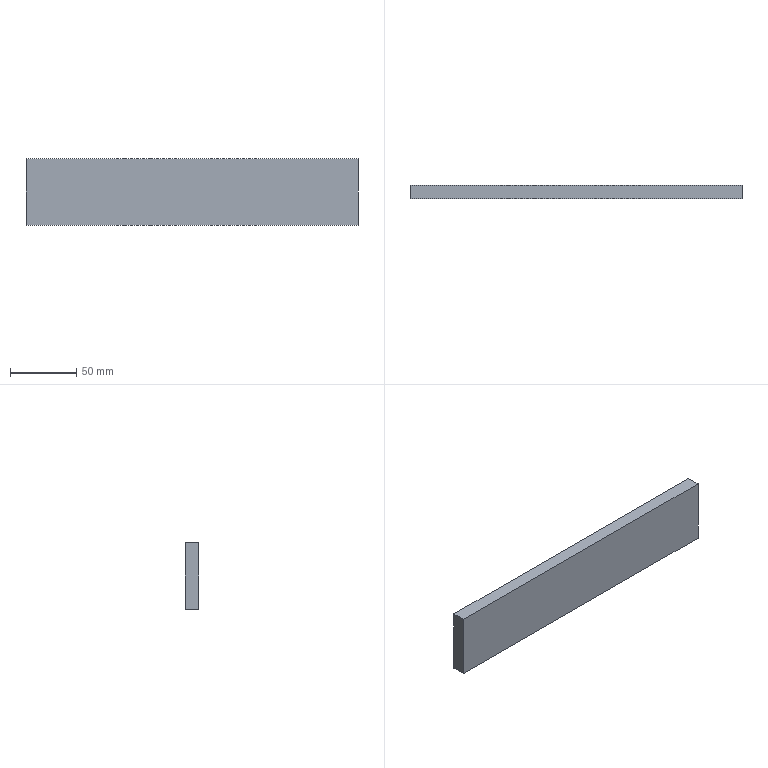Component | NX | FRONT_BLOCK | 1 solid | 6 faces | box 250 x 10 x 50 mm | volume 125000 mm3 | plane 6
STEP:
#1=CARTESIAN_POINT('',(0.,0.,0.));
#2=DIRECTION('',(0.,0.,1.));
#3=DIRECTION('',(1.,0.,0.));
#4=AXIS2_PLACEMENT_3D('',#1,#2,#3);
#5=CARTESIAN_POINT('',(280.662,80.,-20.));
#6=VERTEX_POINT('',#5);
#7=CARTESIAN_POINT('',(280.662,80.,30.));
#8=VERTEX_POINT('',#7);
#9=CARTESIAN_POINT('',(280.662,80.,-20.));
#10=DIRECTION('',(-0.,0.,1.));
#11=VECTOR('',#10,1.);
#12=LINE('',#9,#11);
#13=CARTESIAN_POINT('',(280.662,90.,-20.));
#14=DIRECTION('',(1.,0.,0.));
#15=DIRECTION('',(0.,0.,-1.));
#16=AXIS2_PLACEMENT_3D('',#13,#14,#15);
#17=PLANE('',#16);
#18=CARTESIAN_POINT('',(0.,-10.));
#19=DIRECTION('',(-1.,0.));
#20=VECTOR('',#19,1.);
#21=LINE('',#18,#20);
#22=(GEOMETRIC_REPRESENTATION_CONTEXT(2)PARAMETRIC_REPRESENTATION_CONTEXT()REPRESENTATION_CONTEXT('',''));
#23=DEFINITIONAL_REPRESENTATION('',(#21),#22);
#24=PCURVE('',#17,#23);
#25=CARTESIAN_POINT('',(280.662,80.,-20.));
#26=DIRECTION('',(0.,1.,0.));
#27=DIRECTION('',(1.,0.,0.));
#28=AXIS2_PLACEMENT_3D('',#25,#26,#27);
#29=PLANE('',#28);
#30=CARTESIAN_POINT('',(0.,0.));
#31=DIRECTION('',(-0.,-1.));
#32=VECTOR('',#31,1.);
#33=LINE('',#30,#32);
#34=(GEOMETRIC_REPRESENTATION_CONTEXT(2)PARAMETRIC_REPRESENTATION_CONTEXT()REPRESENTATION_CONTEXT('',''));
#35=DEFINITIONAL_REPRESENTATION('',(#33),#34);
#36=PCURVE('',#29,#35);
#37=SURFACE_CURVE('',#12,(#24,#36),.PCURVE_S1.);
#38=EDGE_CURVE('',#6,#8,#37,.T.);
#39=ORIENTED_EDGE('',*,*,#38,.T.);
#40=CARTESIAN_POINT('',(280.662,90.,30.));
#41=VERTEX_POINT('',#40);
#42=CARTESIAN_POINT('',(280.662,90.,30.));
#43=DIRECTION('',(0.,-1.,0.));
#44=VECTOR('',#43,1.);
#45=LINE('',#42,#44);
#46=CARTESIAN_POINT('',(-50.,0.));
#47=DIRECTION('',(0.,-1.));
#48=VECTOR('',#47,1.);
#49=LINE('',#46,#48);
#50=(GEOMETRIC_REPRESENTATION_CONTEXT(2)PARAMETRIC_REPRESENTATION_CONTEXT()REPRESENTATION_CONTEXT('',''));
#51=DEFINITIONAL_REPRESENTATION('',(#49),#50);
#52=PCURVE('',#17,#51);
#53=CARTESIAN_POINT('',(280.662,90.,30.));
#54=DIRECTION('',(0.,0.,-1.));
#55=DIRECTION('',(0.,1.,0.));
#56=AXIS2_PLACEMENT_3D('',#53,#54,#55);
#57=PLANE('',#56);
#58=CARTESIAN_POINT('',(0.,0.));
#59=DIRECTION('',(-1.,0.));
#60=VECTOR('',#59,1.);
#61=LINE('',#58,#60);
#62=(GEOMETRIC_REPRESENTATION_CONTEXT(2)PARAMETRIC_REPRESENTATION_CONTEXT()REPRESENTATION_CONTEXT('',''));
#63=DEFINITIONAL_REPRESENTATION('',(#61),#62);
#64=PCURVE('',#57,#63);
#65=SURFACE_CURVE('',#45,(#52,#64),.PCURVE_S1.);
#66=EDGE_CURVE('',#41,#8,#65,.T.);
#67=ORIENTED_EDGE('',*,*,#66,.F.);
#68=CARTESIAN_POINT('',(280.662,90.,-20.));
#69=VERTEX_POINT('',#68);
#70=CARTESIAN_POINT('',(280.662,90.,-20.));
#71=DIRECTION('',(-0.,0.,1.));
#72=VECTOR('',#71,1.);
#73=LINE('',#70,#72);
#74=CARTESIAN_POINT('',(0.,0.));
#75=DIRECTION('',(-1.,0.));
#76=VECTOR('',#75,1.);
#77=LINE('',#74,#76);
#78=(GEOMETRIC_REPRESENTATION_CONTEXT(2)PARAMETRIC_REPRESENTATION_CONTEXT()REPRESENTATION_CONTEXT('',''));
#79=DEFINITIONAL_REPRESENTATION('',(#77),#78);
#80=PCURVE('',#17,#79);
#81=CARTESIAN_POINT('',(280.662,90.,-20.));
#82=DIRECTION('',(0.,1.,0.));
#83=DIRECTION('',(1.,0.,0.));
#84=AXIS2_PLACEMENT_3D('',#81,#82,#83);
#85=PLANE('',#84);
#86=CARTESIAN_POINT('',(0.,0.));
#87=DIRECTION('',(-0.,-1.));
#88=VECTOR('',#87,1.);
#89=LINE('',#86,#88);
#90=(GEOMETRIC_REPRESENTATION_CONTEXT(2)PARAMETRIC_REPRESENTATION_CONTEXT()REPRESENTATION_CONTEXT('',''));
#91=DEFINITIONAL_REPRESENTATION('',(#89),#90);
#92=PCURVE('',#85,#91);
#93=SURFACE_CURVE('',#73,(#80,#92),.PCURVE_S1.);
#94=EDGE_CURVE('',#69,#41,#93,.T.);
#95=ORIENTED_EDGE('',*,*,#94,.F.);
#96=CARTESIAN_POINT('',(280.662,90.,-20.));
#97=DIRECTION('',(0.,-1.,0.));
#98=VECTOR('',#97,1.);
#99=LINE('',#96,#98);
#100=CARTESIAN_POINT('',(0.,0.));
#101=DIRECTION('',(0.,-1.));
#102=VECTOR('',#101,1.);
#103=LINE('',#100,#102);
#104=(GEOMETRIC_REPRESENTATION_CONTEXT(2)PARAMETRIC_REPRESENTATION_CONTEXT()REPRESENTATION_CONTEXT('',''));
#105=DEFINITIONAL_REPRESENTATION('',(#103),#104);
#106=PCURVE('',#17,#105);
#107=CARTESIAN_POINT('',(530.662,90.,-20.));
#108=DIRECTION('',(0.,0.,1.));
#109=DIRECTION('',(0.,-1.,0.));
#110=AXIS2_PLACEMENT_3D('',#107,#108,#109);
#111=PLANE('',#110);
#112=CARTESIAN_POINT('',(0.,-250.));
#113=DIRECTION('',(1.,0.));
#114=VECTOR('',#113,1.);
#115=LINE('',#112,#114);
#116=(GEOMETRIC_REPRESENTATION_CONTEXT(2)PARAMETRIC_REPRESENTATION_CONTEXT()REPRESENTATION_CONTEXT('',''));
#117=DEFINITIONAL_REPRESENTATION('',(#115),#116);
#118=PCURVE('',#111,#117);
#119=SURFACE_CURVE('',#99,(#106,#118),.PCURVE_S1.);
#120=EDGE_CURVE('',#69,#6,#119,.T.);
#121=ORIENTED_EDGE('',*,*,#120,.T.);
#122=EDGE_LOOP('',(#39,#67,#95,#121));
#123=FACE_BOUND('',#122,.T.);
#124=ADVANCED_FACE('',(#123),#17,.F.);
#125=CARTESIAN_POINT('',(530.662,80.,30.));
#126=VERTEX_POINT('',#125);
#127=CARTESIAN_POINT('',(280.662,80.,30.));
#128=DIRECTION('',(1.,0.,0.));
#129=VECTOR('',#128,1.);
#130=LINE('',#127,#129);
#131=CARTESIAN_POINT('',(-10.,0.));
#132=DIRECTION('',(0.,1.));
#133=VECTOR('',#132,1.);
#134=LINE('',#131,#133);
#135=(GEOMETRIC_REPRESENTATION_CONTEXT(2)PARAMETRIC_REPRESENTATION_CONTEXT()REPRESENTATION_CONTEXT('',''));
#136=DEFINITIONAL_REPRESENTATION('',(#134),#135);
#137=PCURVE('',#57,#136);
#138=CARTESIAN_POINT('',(0.,-50.));
#139=DIRECTION('',(1.,0.));
#140=VECTOR('',#139,1.);
#141=LINE('',#138,#140);
#142=(GEOMETRIC_REPRESENTATION_CONTEXT(2)PARAMETRIC_REPRESENTATION_CONTEXT()REPRESENTATION_CONTEXT('',''));
#143=DEFINITIONAL_REPRESENTATION('',(#141),#142);
#144=PCURVE('',#29,#143);
#145=SURFACE_CURVE('',#130,(#137,#144),.PCURVE_S1.);
#146=EDGE_CURVE('',#8,#126,#145,.T.);
#147=ORIENTED_EDGE('',*,*,#146,.T.);
#148=CARTESIAN_POINT('',(530.662,90.,30.));
#149=VERTEX_POINT('',#148);
#150=CARTESIAN_POINT('',(530.662,90.,30.));
#151=DIRECTION('',(0.,-1.,0.));
#152=VECTOR('',#151,1.);
#153=LINE('',#150,#152);
#154=CARTESIAN_POINT('',(0.,250.));
#155=DIRECTION('',(-1.,0.));
#156=VECTOR('',#155,1.);
#157=LINE('',#154,#156);
#158=(GEOMETRIC_REPRESENTATION_CONTEXT(2)PARAMETRIC_REPRESENTATION_CONTEXT()REPRESENTATION_CONTEXT('',''));
#159=DEFINITIONAL_REPRESENTATION('',(#157),#158);
#160=PCURVE('',#57,#159);
#161=CARTESIAN_POINT('',(530.662,90.,30.));
#162=DIRECTION('',(-1.,0.,0.));
#163=DIRECTION('',(0.,0.,1.));
#164=AXIS2_PLACEMENT_3D('',#161,#162,#163);
#165=PLANE('',#164);
#166=CARTESIAN_POINT('',(0.,0.));
#167=DIRECTION('',(0.,-1.));
#168=VECTOR('',#167,1.);
#169=LINE('',#166,#168);
#170=(GEOMETRIC_REPRESENTATION_CONTEXT(2)PARAMETRIC_REPRESENTATION_CONTEXT()REPRESENTATION_CONTEXT('',''));
#171=DEFINITIONAL_REPRESENTATION('',(#169),#170);
#172=PCURVE('',#165,#171);
#173=SURFACE_CURVE('',#153,(#160,#172),.PCURVE_S1.);
#174=EDGE_CURVE('',#149,#126,#173,.T.);
#175=ORIENTED_EDGE('',*,*,#174,.F.);
#176=CARTESIAN_POINT('',(280.662,90.,30.));
#177=DIRECTION('',(1.,0.,0.));
#178=VECTOR('',#177,1.);
#179=LINE('',#176,#178);
#180=CARTESIAN_POINT('',(0.,0.));
#181=DIRECTION('',(0.,1.));
#182=VECTOR('',#181,1.);
#183=LINE('',#180,#182);
#184=(GEOMETRIC_REPRESENTATION_CONTEXT(2)PARAMETRIC_REPRESENTATION_CONTEXT()REPRESENTATION_CONTEXT('',''));
#185=DEFINITIONAL_REPRESENTATION('',(#183),#184);
#186=PCURVE('',#57,#185);
#187=CARTESIAN_POINT('',(0.,-50.));
#188=DIRECTION('',(1.,0.));
#189=VECTOR('',#188,1.);
#190=LINE('',#187,#189);
#191=(GEOMETRIC_REPRESENTATION_CONTEXT(2)PARAMETRIC_REPRESENTATION_CONTEXT()REPRESENTATION_CONTEXT('',''));
#192=DEFINITIONAL_REPRESENTATION('',(#190),#191);
#193=PCURVE('',#85,#192);
#194=SURFACE_CURVE('',#179,(#186,#193),.PCURVE_S1.);
#195=EDGE_CURVE('',#41,#149,#194,.T.);
#196=ORIENTED_EDGE('',*,*,#195,.F.);
#197=ORIENTED_EDGE('',*,*,#66,.T.);
#198=EDGE_LOOP('',(#147,#175,#196,#197));
#199=FACE_BOUND('',#198,.T.);
#200=ADVANCED_FACE('',(#199),#57,.F.);
#201=CARTESIAN_POINT('',(530.662,80.,-20.));
#202=VERTEX_POINT('',#201);
#203=CARTESIAN_POINT('',(530.662,80.,30.));
#204=DIRECTION('',(-0.,0.,-1.));
#205=VECTOR('',#204,1.);
#206=LINE('',#203,#205);
#207=CARTESIAN_POINT('',(0.,-10.));
#208=DIRECTION('',(-1.,0.));
#209=VECTOR('',#208,1.);
#210=LINE('',#207,#209);
#211=(GEOMETRIC_REPRESENTATION_CONTEXT(2)PARAMETRIC_REPRESENTATION_CONTEXT()REPRESENTATION_CONTEXT('',''));
#212=DEFINITIONAL_REPRESENTATION('',(#210),#211);
#213=PCURVE('',#165,#212);
#214=CARTESIAN_POINT('',(250.,-50.));
#215=DIRECTION('',(-0.,1.));
#216=VECTOR('',#215,1.);
#217=LINE('',#214,#216);
#218=(GEOMETRIC_REPRESENTATION_CONTEXT(2)PARAMETRIC_REPRESENTATION_CONTEXT()REPRESENTATION_CONTEXT('',''));
#219=DEFINITIONAL_REPRESENTATION('',(#217),#218);
#220=PCURVE('',#29,#219);
#221=SURFACE_CURVE('',#206,(#213,#220),.PCURVE_S1.);
#222=EDGE_CURVE('',#126,#202,#221,.T.);
#223=ORIENTED_EDGE('',*,*,#222,.T.);
#224=CARTESIAN_POINT('',(530.662,90.,-20.));
#225=VERTEX_POINT('',#224);
#226=CARTESIAN_POINT('',(530.662,90.,-20.));
#227=DIRECTION('',(0.,-1.,0.));
#228=VECTOR('',#227,1.);
#229=LINE('',#226,#228);
#230=CARTESIAN_POINT('',(-50.,0.));
#231=DIRECTION('',(0.,-1.));
#232=VECTOR('',#231,1.);
#233=LINE('',#230,#232);
#234=(GEOMETRIC_REPRESENTATION_CONTEXT(2)PARAMETRIC_REPRESENTATION_CONTEXT()REPRESENTATION_CONTEXT('',''));
#235=DEFINITIONAL_REPRESENTATION('',(#233),#234);
#236=PCURVE('',#165,#235);
#237=CARTESIAN_POINT('',(0.,0.));
#238=DIRECTION('',(1.,0.));
#239=VECTOR('',#238,1.);
#240=LINE('',#237,#239);
#241=(GEOMETRIC_REPRESENTATION_CONTEXT(2)PARAMETRIC_REPRESENTATION_CONTEXT()REPRESENTATION_CONTEXT('',''));
#242=DEFINITIONAL_REPRESENTATION('',(#240),#241);
#243=PCURVE('',#111,#242);
#244=SURFACE_CURVE('',#229,(#236,#243),.PCURVE_S1.);
#245=EDGE_CURVE('',#225,#202,#244,.T.);
#246=ORIENTED_EDGE('',*,*,#245,.F.);
#247=CARTESIAN_POINT('',(530.662,90.,30.));
#248=DIRECTION('',(-0.,0.,-1.));
#249=VECTOR('',#248,1.);
#250=LINE('',#247,#249);
#251=CARTESIAN_POINT('',(0.,0.));
#252=DIRECTION('',(-1.,0.));
#253=VECTOR('',#252,1.);
#254=LINE('',#251,#253);
#255=(GEOMETRIC_REPRESENTATION_CONTEXT(2)PARAMETRIC_REPRESENTATION_CONTEXT()REPRESENTATION_CONTEXT('',''));
#256=DEFINITIONAL_REPRESENTATION('',(#254),#255);
#257=PCURVE('',#165,#256);
#258=CARTESIAN_POINT('',(250.,-50.));
#259=DIRECTION('',(-0.,1.));
#260=VECTOR('',#259,1.);
#261=LINE('',#258,#260);
#262=(GEOMETRIC_REPRESENTATION_CONTEXT(2)PARAMETRIC_REPRESENTATION_CONTEXT()REPRESENTATION_CONTEXT('',''));
#263=DEFINITIONAL_REPRESENTATION('',(#261),#262);
#264=PCURVE('',#85,#263);
#265=SURFACE_CURVE('',#250,(#257,#264),.PCURVE_S1.);
#266=EDGE_CURVE('',#149,#225,#265,.T.);
#267=ORIENTED_EDGE('',*,*,#266,.F.);
#268=ORIENTED_EDGE('',*,*,#174,.T.);
#269=EDGE_LOOP('',(#223,#246,#267,#268));
#270=FACE_BOUND('',#269,.T.);
#271=ADVANCED_FACE('',(#270),#165,.F.);
#272=CARTESIAN_POINT('',(530.662,80.,-20.));
#273=DIRECTION('',(-1.,0.,0.));
#274=VECTOR('',#273,1.);
#275=LINE('',#272,#274);
#276=CARTESIAN_POINT('',(10.,0.));
#277=DIRECTION('',(0.,-1.));
#278=VECTOR('',#277,1.);
#279=LINE('',#276,#278);
#280=(GEOMETRIC_REPRESENTATION_CONTEXT(2)PARAMETRIC_REPRESENTATION_CONTEXT()REPRESENTATION_CONTEXT('',''));
#281=DEFINITIONAL_REPRESENTATION('',(#279),#280);
#282=PCURVE('',#111,#281);
#283=CARTESIAN_POINT('',(250.,0.));
#284=DIRECTION('',(-1.,0.));
#285=VECTOR('',#284,1.);
#286=LINE('',#283,#285);
#287=(GEOMETRIC_REPRESENTATION_CONTEXT(2)PARAMETRIC_REPRESENTATION_CONTEXT()REPRESENTATION_CONTEXT('',''));
#288=DEFINITIONAL_REPRESENTATION('',(#286),#287);
#289=PCURVE('',#29,#288);
#290=SURFACE_CURVE('',#275,(#282,#289),.PCURVE_S1.);
#291=EDGE_CURVE('',#202,#6,#290,.T.);
#292=ORIENTED_EDGE('',*,*,#291,.T.);
#293=ORIENTED_EDGE('',*,*,#120,.F.);
#294=CARTESIAN_POINT('',(530.662,90.,-20.));
#295=DIRECTION('',(-1.,0.,0.));
#296=VECTOR('',#295,1.);
#297=LINE('',#294,#296);
#298=CARTESIAN_POINT('',(0.,0.));
#299=DIRECTION('',(0.,-1.));
#300=VECTOR('',#299,1.);
#301=LINE('',#298,#300);
#302=(GEOMETRIC_REPRESENTATION_CONTEXT(2)PARAMETRIC_REPRESENTATION_CONTEXT()REPRESENTATION_CONTEXT('',''));
#303=DEFINITIONAL_REPRESENTATION('',(#301),#302);
#304=PCURVE('',#111,#303);
#305=CARTESIAN_POINT('',(250.,0.));
#306=DIRECTION('',(-1.,0.));
#307=VECTOR('',#306,1.);
#308=LINE('',#305,#307);
#309=(GEOMETRIC_REPRESENTATION_CONTEXT(2)PARAMETRIC_REPRESENTATION_CONTEXT()REPRESENTATION_CONTEXT('',''));
#310=DEFINITIONAL_REPRESENTATION('',(#308),#309);
#311=PCURVE('',#85,#310);
#312=SURFACE_CURVE('',#297,(#304,#311),.PCURVE_S1.);
#313=EDGE_CURVE('',#225,#69,#312,.T.);
#314=ORIENTED_EDGE('',*,*,#313,.F.);
#315=ORIENTED_EDGE('',*,*,#245,.T.);
#316=EDGE_LOOP('',(#292,#293,#314,#315));
#317=FACE_BOUND('',#316,.T.);
#318=ADVANCED_FACE('',(#317),#111,.F.);
#319=ORIENTED_EDGE('',*,*,#94,.T.);
#320=ORIENTED_EDGE('',*,*,#195,.T.);
#321=ORIENTED_EDGE('',*,*,#266,.T.);
#322=ORIENTED_EDGE('',*,*,#313,.T.);
#323=EDGE_LOOP('',(#319,#320,#321,#322));
#324=FACE_BOUND('',#323,.T.);
#325=ADVANCED_FACE('',(#324),#85,.T.);
#326=ORIENTED_EDGE('',*,*,#38,.F.);
#327=ORIENTED_EDGE('',*,*,#291,.F.);
#328=ORIENTED_EDGE('',*,*,#222,.F.);
#329=ORIENTED_EDGE('',*,*,#146,.F.);
#330=EDGE_LOOP('',(#326,#327,#328,#329));
#331=FACE_BOUND('',#330,.T.);
#332=ADVANCED_FACE('',(#331),#29,.F.);
#333=CLOSED_SHELL('',(#124,#200,#271,#318,#325,#332));
#334=MANIFOLD_SOLID_BREP('',#333);
#335=(LENGTH_UNIT()NAMED_UNIT(*)SI_UNIT(.MILLI.,.METRE.));
#336=UNCERTAINTY_MEASURE_WITH_UNIT(LENGTH_MEASURE(0.0000001),#335,'','');
#337=(NAMED_UNIT(*)PLANE_ANGLE_UNIT()SI_UNIT($,.RADIAN.));
#338=(NAMED_UNIT(*)SI_UNIT($,.STERADIAN.)SOLID_ANGLE_UNIT());
#339=(GEOMETRIC_REPRESENTATION_CONTEXT(3)GLOBAL_UNCERTAINTY_ASSIGNED_CONTEXT((#336))GLOBAL_UNIT_ASSIGNED_CONTEXT((#335,#337,#338))REPRESENTATION_CONTEXT('',''));
#340=ADVANCED_BREP_SHAPE_REPRESENTATION('',(#4,#334),#339);